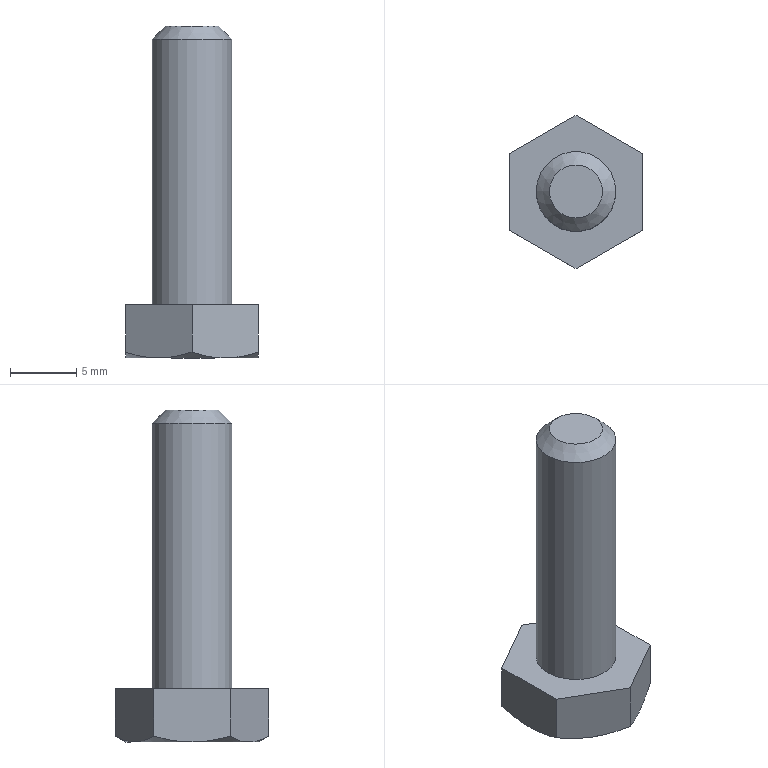Component | NX | BOLT_M6_2 | 1 solid | 17 faces | volume 931 mm3 | plane 9 | cone 7 | cylinder 1 | commonest cylinder face diameters 6 x1